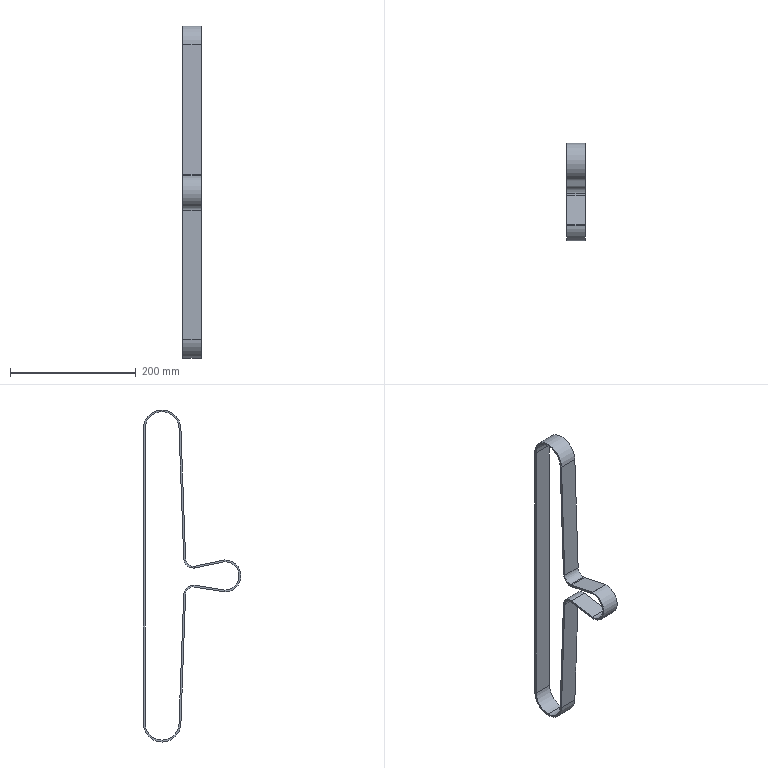Component | SolidWorks | Belt-1 | 1 solid | 28 faces | box 30 x 155.5 x 528 mm | volume 115040 mm3 | cylinder 16 | plane 12 | commonest cylinder face diameters 31.04 x3 54 x3 60 x3 25.04 x3 51 x3 45 x1
build123d program:
from build123d import *

# Parameters (mm, degrees)
BOSS_EXTRUDE1_DEPTH = 15


with BuildPart() as part:
    # Sketch1 → Boss-Extrude1 (new, symmetric)
    with BuildSketch(Plane.XY):
        with BuildLine():
            Line((-104.56, 30), (363.44, 30))
            ThreePointArc((363.44, 30), (393.44, 0.03848), (363.517, -30))
            Line((363.517, -30), (156.987, -37.488))
            ThreePointArc((156.987, -37.488), (147.591, -42.27), (145.179, -52.533))
            Line((145.179, -52.533), (154.939, -99.785))
            ThreePointArc((154.939, -99.785), (129.473, -125.5), (103.941, -99.851))
            Line((103.941, -99.851), (111.795, -52.029))
            ThreePointArc((111.795, -52.029), (109.13, -42.072), (99.898, -37.488))
            Line((99.898, -37.488), (-104.639, -30))
            ThreePointArc((-104.639, -30), (-134.56, 0.03959), (-104.56, 30))
        make_face()
        with BuildLine():
            Line((-104.56, 27), (363.44, 27))
            ThreePointArc((363.44, 27), (390.44, 0), (363.44, -27))
            Line((363.44, -27), (156.878, -34.49))
            ThreePointArc((156.878, -34.49), (145.229, -40.42), (142.242, -53.146))
            Line((142.242, -53.146), (151.94, -100))
            ThreePointArc((151.94, -100), (129.44, -122.5), (106.94, -100))
            Line((106.94, -100), (114.754, -52.52))
            ThreePointArc((114.754, -52.52), (111.454, -40.174), (100.008, -34.49))
            Line((100.008, -34.49), (-104.56, -27))
            ThreePointArc((-104.56, -27), (-131.56, 0), (-104.56, 27))
        make_face(mode=Mode.SUBTRACT)
    extrude(amount=BOSS_EXTRUDE1_DEPTH, both=True)


solid = part.part

# Placed as in the assembly
solid = solid.moved(Location((-0.0005, 4.001, -329.44), (0, -90, 0)))
STEP:
#1=COLOUR_RGB('',0.7922,0.8196,0.9333);
#2=FILL_AREA_STYLE_COLOUR('',#1);
#3=FILL_AREA_STYLE('',(#2));
#4=SURFACE_STYLE_FILL_AREA(#3);
#5=SURFACE_SIDE_STYLE('',(#4));
#6=SURFACE_STYLE_USAGE(.BOTH.,#5);
#7=PRESENTATION_STYLE_ASSIGNMENT((#6));
#8=CARTESIAN_POINT('',(-0.5906,-1.935,-7.37));
#9=VERTEX_POINT('',#8);
#10=CARTESIAN_POINT('',(-0.5906,-1.811,-7.383));
#11=VERTEX_POINT('',#10);
#12=CARTESIAN_POINT('',(-0.5906,-1.811,-6.772));
#13=DIRECTION('',(1.,0.,0.));
#14=DIRECTION('',(0.,0.,-1.));
#15=AXIS2_PLACEMENT_3D('',#12,#13,#14);
#16=CIRCLE('',#15,0.611);
#17=EDGE_CURVE('',#9,#11,#16,.T.);
#18=ORIENTED_EDGE('',*,*,#17,.T.);
#19=CARTESIAN_POINT('',(0.5905,-1.811,-7.383));
#20=VERTEX_POINT('',#19);
#21=CARTESIAN_POINT('',(-0.5906,-1.811,-7.383));
#22=DIRECTION('',(1.,0.,0.));
#23=VECTOR('',#22,39.37);
#24=LINE('',#21,#23);
#25=EDGE_CURVE('',#11,#20,#24,.T.);
#26=ORIENTED_EDGE('',*,*,#25,.T.);
#27=CARTESIAN_POINT('',(0.5905,-1.935,-7.37));
#28=VERTEX_POINT('',#27);
#29=CARTESIAN_POINT('',(0.5905,-1.811,-6.772));
#30=DIRECTION('',(1.,0.,0.));
#31=DIRECTION('',(0.,0.,-1.));
#32=AXIS2_PLACEMENT_3D('',#29,#30,#31);
#33=CIRCLE('',#32,0.611);
#34=EDGE_CURVE('',#28,#20,#33,.T.);
#35=ORIENTED_EDGE('',*,*,#34,.F.);
#36=CARTESIAN_POINT('',(-0.5906,-1.935,-7.37));
#37=DIRECTION('',(1.,0.,0.));
#38=VECTOR('',#37,39.37);
#39=LINE('',#36,#38);
#40=EDGE_CURVE('',#9,#28,#39,.T.);
#41=ORIENTED_EDGE('',*,*,#40,.F.);
#42=EDGE_LOOP('',(#18,#26,#35,#41));
#43=FACE_OUTER_BOUND('',#42,.T.);
#44=CARTESIAN_POINT('',(-0.5906,-1.811,-6.772));
#45=DIRECTION('',(1.,0.,0.));
#46=DIRECTION('',(0.,0.,-1.));
#47=AXIS2_PLACEMENT_3D('',#44,#45,#46);
#48=CYLINDRICAL_SURFACE('',#47,0.611);
#49=ADVANCED_FACE('',(#43),#48,.T.);
#50=CARTESIAN_POINT('',(-0.5906,1.221,-17.087));
#51=VERTEX_POINT('',#50);
#52=CARTESIAN_POINT('',(-0.5906,0.1575,-18.15));
#53=VERTEX_POINT('',#52);
#54=CARTESIAN_POINT('',(-0.5906,0.1575,-17.087));
#55=DIRECTION('',(-1.,0.,0.));
#56=DIRECTION('',(0.,0.,1.));
#57=AXIS2_PLACEMENT_3D('',#54,#55,#56);
#58=CIRCLE('',#57,1.063);
#59=EDGE_CURVE('',#51,#53,#58,.T.);
#60=ORIENTED_EDGE('',*,*,#59,.T.);
#61=CARTESIAN_POINT('',(0.5905,0.1575,-18.15));
#62=VERTEX_POINT('',#61);
#63=CARTESIAN_POINT('',(-0.5906,0.1575,-18.15));
#64=DIRECTION('',(1.,0.,0.));
#65=VECTOR('',#64,39.37);
#66=LINE('',#63,#65);
#67=EDGE_CURVE('',#53,#62,#66,.T.);
#68=ORIENTED_EDGE('',*,*,#67,.T.);
#69=CARTESIAN_POINT('',(0.5905,1.221,-17.087));
#70=VERTEX_POINT('',#69);
#71=CARTESIAN_POINT('',(0.5905,0.1575,-17.087));
#72=DIRECTION('',(-1.,0.,0.));
#73=DIRECTION('',(0.,0.,1.));
#74=AXIS2_PLACEMENT_3D('',#71,#72,#73);
#75=CIRCLE('',#74,1.063);
#76=EDGE_CURVE('',#70,#62,#75,.T.);
#77=ORIENTED_EDGE('',*,*,#76,.F.);
#78=CARTESIAN_POINT('',(-0.5906,1.221,-17.087));
#79=DIRECTION('',(1.,0.,0.));
#80=VECTOR('',#79,39.37);
#81=LINE('',#78,#80);
#82=EDGE_CURVE('',#51,#70,#81,.T.);
#83=ORIENTED_EDGE('',*,*,#82,.F.);
#84=EDGE_LOOP('',(#60,#68,#77,#83));
#85=FACE_OUTER_BOUND('',#84,.T.);
#86=CARTESIAN_POINT('',(-0.5906,0.1575,-17.087));
#87=DIRECTION('',(1.,0.,0.));
#88=DIRECTION('',(0.,0.,-1.));
#89=AXIS2_PLACEMENT_3D('',#86,#87,#88);
#90=CYLINDRICAL_SURFACE('',#89,1.063);
#91=ADVANCED_FACE('',(#85),#90,.F.);
#92=CARTESIAN_POINT('',(-0.5906,0.1575,-18.268));
#93=VERTEX_POINT('',#92);
#94=CARTESIAN_POINT('',(-0.5906,-1.024,-17.09));
#95=VERTEX_POINT('',#94);
#96=CARTESIAN_POINT('',(-0.5906,0.1575,-17.087));
#97=DIRECTION('',(-1.,0.,0.));
#98=DIRECTION('',(0.,0.,1.));
#99=AXIS2_PLACEMENT_3D('',#96,#97,#98);
#100=CIRCLE('',#99,1.181);
#101=EDGE_CURVE('',#93,#95,#100,.T.);
#102=ORIENTED_EDGE('',*,*,#101,.F.);
#103=CARTESIAN_POINT('',(0.5905,0.1575,-18.268));
#104=VERTEX_POINT('',#103);
#105=CARTESIAN_POINT('',(-0.5906,0.1575,-18.268));
#106=DIRECTION('',(1.,0.,0.));
#107=VECTOR('',#106,39.37);
#108=LINE('',#105,#107);
#109=EDGE_CURVE('',#93,#104,#108,.T.);
#110=ORIENTED_EDGE('',*,*,#109,.T.);
#111=CARTESIAN_POINT('',(0.5905,-1.024,-17.09));
#112=VERTEX_POINT('',#111);
#113=CARTESIAN_POINT('',(0.5905,0.1575,-17.087));
#114=DIRECTION('',(-1.,0.,0.));
#115=DIRECTION('',(0.,0.,1.));
#116=AXIS2_PLACEMENT_3D('',#113,#114,#115);
#117=CIRCLE('',#116,1.181);
#118=EDGE_CURVE('',#104,#112,#117,.T.);
#119=ORIENTED_EDGE('',*,*,#118,.T.);
#120=CARTESIAN_POINT('',(-0.5906,-1.024,-17.09));
#121=DIRECTION('',(1.,0.,0.));
#122=VECTOR('',#121,39.37);
#123=LINE('',#120,#122);
#124=EDGE_CURVE('',#95,#112,#123,.T.);
#125=ORIENTED_EDGE('',*,*,#124,.F.);
#126=EDGE_LOOP('',(#102,#110,#119,#125));
#127=FACE_OUTER_BOUND('',#126,.T.);
#128=CARTESIAN_POINT('',(-0.5906,0.1575,-17.087));
#129=DIRECTION('',(1.,0.,0.));
#130=DIRECTION('',(0.,0.,-1.));
#131=AXIS2_PLACEMENT_3D('',#128,#129,#130);
#132=CYLINDRICAL_SURFACE('',#131,1.181);
#133=ADVANCED_FACE('',(#127),#132,.T.);
#134=CARTESIAN_POINT('',(-0.5906,-1.811,-7.265));
#135=VERTEX_POINT('',#134);
#136=CARTESIAN_POINT('',(-0.5906,-1.318,-6.79));
#137=VERTEX_POINT('',#136);
#138=CARTESIAN_POINT('',(-0.5906,-1.811,-6.772));
#139=DIRECTION('',(1.,0.,0.));
#140=DIRECTION('',(0.,0.,-1.));
#141=AXIS2_PLACEMENT_3D('',#138,#139,#140);
#142=CIRCLE('',#141,0.4929);
#143=EDGE_CURVE('',#135,#137,#142,.T.);
#144=ORIENTED_EDGE('',*,*,#143,.F.);
#145=CARTESIAN_POINT('',(0.5905,-1.811,-7.265));
#146=VERTEX_POINT('',#145);
#147=CARTESIAN_POINT('',(-0.5906,-1.811,-7.265));
#148=DIRECTION('',(1.,0.,0.));
#149=VECTOR('',#148,39.37);
#150=LINE('',#147,#149);
#151=EDGE_CURVE('',#135,#146,#150,.T.);
#152=ORIENTED_EDGE('',*,*,#151,.T.);
#153=CARTESIAN_POINT('',(0.5905,-1.318,-6.79));
#154=VERTEX_POINT('',#153);
#155=CARTESIAN_POINT('',(0.5905,-1.811,-6.772));
#156=DIRECTION('',(1.,0.,0.));
#157=DIRECTION('',(0.,0.,-1.));
#158=AXIS2_PLACEMENT_3D('',#155,#156,#157);
#159=CIRCLE('',#158,0.4929);
#160=EDGE_CURVE('',#146,#154,#159,.T.);
#161=ORIENTED_EDGE('',*,*,#160,.T.);
#162=CARTESIAN_POINT('',(-0.5906,-1.318,-6.79));
#163=DIRECTION('',(1.,0.,0.));
#164=VECTOR('',#163,39.37);
#165=LINE('',#162,#164);
#166=EDGE_CURVE('',#137,#154,#165,.T.);
#167=ORIENTED_EDGE('',*,*,#166,.F.);
#168=EDGE_LOOP('',(#144,#152,#161,#167));
#169=FACE_OUTER_BOUND('',#168,.T.);
#170=CARTESIAN_POINT('',(-0.5906,-1.811,-6.772));
#171=DIRECTION('',(1.,0.,0.));
#172=DIRECTION('',(0.,0.,-1.));
#173=AXIS2_PLACEMENT_3D('',#170,#171,#172);
#174=CYLINDRICAL_SURFACE('',#173,0.4929);
#175=ADVANCED_FACE('',(#169),#174,.F.);
#176=CARTESIAN_POINT('',(-0.5906,-3.779,-6.87));
#177=VERTEX_POINT('',#176);
#178=CARTESIAN_POINT('',(-0.5906,-3.771,-6.87));
#179=VERTEX_POINT('',#178);
#180=CARTESIAN_POINT('',(-0.5906,-3.779,-7.874));
#181=DIRECTION('',(-1.,0.,0.));
#182=DIRECTION('',(0.,0.,1.));
#183=AXIS2_PLACEMENT_3D('',#180,#181,#182);
#184=CIRCLE('',#183,1.004);
#185=EDGE_CURVE('',#177,#179,#184,.T.);
#186=ORIENTED_EDGE('',*,*,#185,.F.);
#187=CARTESIAN_POINT('',(0.5905,-3.779,-6.87));
#188=VERTEX_POINT('',#187);
#189=CARTESIAN_POINT('',(-0.5906,-3.779,-6.87));
#190=DIRECTION('',(1.,0.,0.));
#191=VECTOR('',#190,39.37);
#192=LINE('',#189,#191);
#193=EDGE_CURVE('',#177,#188,#192,.T.);
#194=ORIENTED_EDGE('',*,*,#193,.T.);
#195=CARTESIAN_POINT('',(0.5905,-3.771,-6.87));
#196=VERTEX_POINT('',#195);
#197=CARTESIAN_POINT('',(0.5905,-3.779,-7.874));
#198=DIRECTION('',(-1.,0.,0.));
#199=DIRECTION('',(0.,0.,1.));
#200=AXIS2_PLACEMENT_3D('',#197,#198,#199);
#201=CIRCLE('',#200,1.004);
#202=EDGE_CURVE('',#188,#196,#201,.T.);
#203=ORIENTED_EDGE('',*,*,#202,.T.);
#204=CARTESIAN_POINT('',(-0.5906,-3.771,-6.87));
#205=DIRECTION('',(1.,0.,0.));
#206=VECTOR('',#205,39.37);
#207=LINE('',#204,#206);
#208=EDGE_CURVE('',#179,#196,#207,.T.);
#209=ORIENTED_EDGE('',*,*,#208,.F.);
#210=EDGE_LOOP('',(#186,#194,#203,#209));
#211=FACE_OUTER_BOUND('',#210,.T.);
#212=CARTESIAN_POINT('',(-0.5906,-3.779,-7.874));
#213=DIRECTION('',(1.,0.,0.));
#214=DIRECTION('',(0.,0.,-1.));
#215=AXIS2_PLACEMENT_3D('',#212,#213,#214);
#216=CYLINDRICAL_SURFACE('',#215,1.004);
#217=ADVANCED_FACE('',(#211),#216,.T.);
#218=ORIENTED_EDGE('',*,*,#193,.F.);
#219=CARTESIAN_POINT('',(-0.5906,-3.779,-8.878));
#220=VERTEX_POINT('',#219);
#221=CARTESIAN_POINT('',(-0.5906,-3.779,-7.874));
#222=DIRECTION('',(-1.,0.,0.));
#223=DIRECTION('',(0.,0.,1.));
#224=AXIS2_PLACEMENT_3D('',#221,#222,#223);
#225=CIRCLE('',#224,1.004);
#226=EDGE_CURVE('',#220,#177,#225,.T.);
#227=ORIENTED_EDGE('',*,*,#226,.F.);
#228=CARTESIAN_POINT('',(0.5905,-3.779,-8.878));
#229=VERTEX_POINT('',#228);
#230=CARTESIAN_POINT('',(-0.5906,-3.779,-8.878));
#231=DIRECTION('',(1.,0.,0.));
#232=VECTOR('',#231,39.37);
#233=LINE('',#230,#232);
#234=EDGE_CURVE('',#220,#229,#233,.T.);
#235=ORIENTED_EDGE('',*,*,#234,.T.);
#236=CARTESIAN_POINT('',(0.5905,-3.779,-7.874));
#237=DIRECTION('',(-1.,0.,0.));
#238=DIRECTION('',(0.,0.,1.));
#239=AXIS2_PLACEMENT_3D('',#236,#237,#238);
#240=CIRCLE('',#239,1.004);
#241=EDGE_CURVE('',#229,#188,#240,.T.);
#242=ORIENTED_EDGE('',*,*,#241,.T.);
#243=EDGE_LOOP('',(#218,#227,#235,#242));
#244=FACE_OUTER_BOUND('',#243,.T.);
#245=CARTESIAN_POINT('',(-0.5906,-3.779,-7.874));
#246=DIRECTION('',(1.,0.,0.));
#247=DIRECTION('',(0.,0.,-1.));
#248=AXIS2_PLACEMENT_3D('',#245,#246,#247);
#249=CYLINDRICAL_SURFACE('',#248,1.004);
#250=ADVANCED_FACE('',(#244),#249,.T.);
#251=CARTESIAN_POINT('',(-0.5906,-3.774,-8.878));
#252=VERTEX_POINT('',#251);
#253=CARTESIAN_POINT('',(-0.5906,-3.779,-7.874));
#254=DIRECTION('',(-1.,0.,0.));
#255=DIRECTION('',(0.,0.,1.));
#256=AXIS2_PLACEMENT_3D('',#253,#254,#255);
#257=CIRCLE('',#256,1.004);
#258=EDGE_CURVE('',#252,#220,#257,.T.);
#259=ORIENTED_EDGE('',*,*,#258,.T.);
#260=ORIENTED_EDGE('',*,*,#226,.T.);
#261=ORIENTED_EDGE('',*,*,#185,.T.);
#262=CARTESIAN_POINT('',(-0.5906,-1.911,-7.254));
#263=VERTEX_POINT('',#262);
#264=CARTESIAN_POINT('',(-0.5906,-3.771,-6.87));
#265=DIRECTION('',(0.,0.9793,-0.2023));
#266=VECTOR('',#265,39.37);
#267=LINE('',#264,#266);
#268=EDGE_CURVE('',#179,#263,#267,.T.);
#269=ORIENTED_EDGE('',*,*,#268,.T.);
#270=CARTESIAN_POINT('',(-0.5906,-1.811,-6.772));
#271=DIRECTION('',(1.,0.,0.));
#272=DIRECTION('',(0.,0.,-1.));
#273=AXIS2_PLACEMENT_3D('',#270,#271,#272);
#274=CIRCLE('',#273,0.4929);
#275=EDGE_CURVE('',#263,#135,#274,.T.);
#276=ORIENTED_EDGE('',*,*,#275,.T.);
#277=ORIENTED_EDGE('',*,*,#143,.T.);
#278=CARTESIAN_POINT('',(-0.5906,-1.024,1.342));
#279=VERTEX_POINT('',#278);
#280=CARTESIAN_POINT('',(-0.5906,-1.024,1.342));
#281=DIRECTION('',(0.,0.03623,0.9993));
#282=VECTOR('',#281,39.37);
#283=LINE('',#280,#282);
#284=EDGE_CURVE('',#137,#279,#283,.T.);
#285=ORIENTED_EDGE('',*,*,#284,.T.);
#286=CARTESIAN_POINT('',(-0.5906,1.339,1.339));
#287=VERTEX_POINT('',#286);
#288=CARTESIAN_POINT('',(-0.5906,0.1575,1.339));
#289=DIRECTION('',(-1.,0.,0.));
#290=DIRECTION('',(0.,0.,-1.));
#291=AXIS2_PLACEMENT_3D('',#288,#289,#290);
#292=CIRCLE('',#291,1.181);
#293=EDGE_CURVE('',#279,#287,#292,.T.);
#294=ORIENTED_EDGE('',*,*,#293,.T.);
#295=CARTESIAN_POINT('',(-0.5906,1.339,-17.087));
#296=VERTEX_POINT('',#295);
#297=CARTESIAN_POINT('',(-0.5906,1.339,-17.087));
#298=DIRECTION('',(0.,-0.,-1.));
#299=VECTOR('',#298,39.37);
#300=LINE('',#297,#299);
#301=EDGE_CURVE('',#287,#296,#300,.T.);
#302=ORIENTED_EDGE('',*,*,#301,.T.);
#303=CARTESIAN_POINT('',(-0.5906,0.1575,-17.087));
#304=DIRECTION('',(-1.,0.,0.));
#305=DIRECTION('',(0.,0.,1.));
#306=AXIS2_PLACEMENT_3D('',#303,#304,#305);
#307=CIRCLE('',#306,1.181);
#308=EDGE_CURVE('',#296,#93,#307,.T.);
#309=ORIENTED_EDGE('',*,*,#308,.T.);
#310=ORIENTED_EDGE('',*,*,#101,.T.);
#311=CARTESIAN_POINT('',(-0.5906,-1.318,-9.037));
#312=VERTEX_POINT('',#311);
#313=CARTESIAN_POINT('',(-0.5906,-1.024,-17.09));
#314=DIRECTION('',(0.,-0.03659,0.9993));
#315=VECTOR('',#314,39.37);
#316=LINE('',#313,#315);
#317=EDGE_CURVE('',#95,#312,#316,.T.);
#318=ORIENTED_EDGE('',*,*,#317,.T.);
#319=CARTESIAN_POINT('',(-0.5906,-1.891,-8.569));
#320=VERTEX_POINT('',#319);
#321=CARTESIAN_POINT('',(-0.5906,-1.811,-9.055));
#322=DIRECTION('',(1.,0.,0.));
#323=DIRECTION('',(0.,0.,-1.));
#324=AXIS2_PLACEMENT_3D('',#321,#322,#323);
#325=CIRCLE('',#324,0.4929);
#326=EDGE_CURVE('',#312,#320,#325,.T.);
#327=ORIENTED_EDGE('',*,*,#326,.T.);
#328=CARTESIAN_POINT('',(-0.5906,-3.774,-8.878));
#329=DIRECTION('',(0.,-0.9868,-0.1621));
#330=VECTOR('',#329,39.37);
#331=LINE('',#328,#330);
#332=EDGE_CURVE('',#320,#252,#331,.T.);
#333=ORIENTED_EDGE('',*,*,#332,.T.);
#334=EDGE_LOOP('',(#259,#260,#261,#269,#276,#277,#285,#294,#302,#309,#310,#318,#327,#333));
#335=FACE_OUTER_BOUND('',#334,.T.);
#336=CARTESIAN_POINT('',(-0.5906,-0.9055,-17.087));
#337=VERTEX_POINT('',#336);
#338=CARTESIAN_POINT('',(-0.5906,-1.2,-9.033));
#339=VERTEX_POINT('',#338);
#340=CARTESIAN_POINT('',(-0.5906,-0.9055,-17.087));
#341=DIRECTION('',(0.,-0.03659,0.9993));
#342=VECTOR('',#341,39.37);
#343=LINE('',#340,#342);
#344=EDGE_CURVE('',#337,#339,#343,.T.);
#345=ORIENTED_EDGE('',*,*,#344,.F.);
#346=CARTESIAN_POINT('',(-0.5906,0.1575,-17.087));
#347=DIRECTION('',(-1.,0.,0.));
#348=DIRECTION('',(0.,0.,1.));
#349=AXIS2_PLACEMENT_3D('',#346,#347,#348);
#350=CIRCLE('',#349,1.063);
#351=EDGE_CURVE('',#53,#337,#350,.T.);
#352=ORIENTED_EDGE('',*,*,#351,.F.);
#353=ORIENTED_EDGE('',*,*,#59,.F.);
#354=CARTESIAN_POINT('',(-0.5906,1.221,1.339));
#355=VERTEX_POINT('',#354);
#356=CARTESIAN_POINT('',(-0.5906,1.221,-17.087));
#357=DIRECTION('',(0.,0.,-1.));
#358=VECTOR('',#357,39.37);
#359=LINE('',#356,#358);
#360=EDGE_CURVE('',#355,#51,#359,.T.);
#361=ORIENTED_EDGE('',*,*,#360,.F.);
#362=CARTESIAN_POINT('',(-0.5906,-0.9055,1.339));
#363=VERTEX_POINT('',#362);
#364=CARTESIAN_POINT('',(-0.5906,0.1575,1.339));
#365=DIRECTION('',(-1.,0.,0.));
#366=DIRECTION('',(0.,0.,-1.));
#367=AXIS2_PLACEMENT_3D('',#364,#365,#366);
#368=CIRCLE('',#367,1.063);
#369=EDGE_CURVE('',#363,#355,#368,.T.);
#370=ORIENTED_EDGE('',*,*,#369,.F.);
#371=CARTESIAN_POINT('',(-0.5906,-1.2,-6.794));
#372=VERTEX_POINT('',#371);
#373=CARTESIAN_POINT('',(-0.5906,-0.9055,1.339));
#374=DIRECTION('',(0.,0.03624,0.9993));
#375=VECTOR('',#374,39.37);
#376=LINE('',#373,#375);
#377=EDGE_CURVE('',#372,#363,#376,.T.);
#378=ORIENTED_EDGE('',*,*,#377,.F.);
#379=CARTESIAN_POINT('',(-0.5906,-1.811,-6.772));
#380=DIRECTION('',(1.,0.,0.));
#381=DIRECTION('',(0.,0.,-1.));
#382=AXIS2_PLACEMENT_3D('',#379,#380,#381);
#383=CIRCLE('',#382,0.611);
#384=EDGE_CURVE('',#11,#372,#383,.T.);
#385=ORIENTED_EDGE('',*,*,#384,.F.);
#386=ORIENTED_EDGE('',*,*,#17,.F.);
#387=CARTESIAN_POINT('',(-0.5906,-3.779,-6.988));
#388=VERTEX_POINT('',#387);
#389=CARTESIAN_POINT('',(-0.5906,-3.779,-6.988));
#390=DIRECTION('',(0.,0.9792,-0.2027));
#391=VECTOR('',#390,39.37);
#392=LINE('',#389,#391);
#393=EDGE_CURVE('',#388,#9,#392,.T.);
#394=ORIENTED_EDGE('',*,*,#393,.F.);
#395=CARTESIAN_POINT('',(-0.5906,-3.779,-8.76));
#396=VERTEX_POINT('',#395);
#397=CARTESIAN_POINT('',(-0.5906,-3.779,-7.874));
#398=DIRECTION('',(-1.,0.,0.));
#399=DIRECTION('',(0.,0.,1.));
#400=AXIS2_PLACEMENT_3D('',#397,#398,#399);
#401=CIRCLE('',#400,0.8858);
#402=EDGE_CURVE('',#396,#388,#401,.T.);
#403=ORIENTED_EDGE('',*,*,#402,.F.);
#404=CARTESIAN_POINT('',(-0.5906,-1.91,-8.452));
#405=VERTEX_POINT('',#404);
#406=CARTESIAN_POINT('',(-0.5906,-3.779,-8.76));
#407=DIRECTION('',(0.,-0.9867,-0.1624));
#408=VECTOR('',#407,39.37);
#409=LINE('',#406,#408);
#410=EDGE_CURVE('',#405,#396,#409,.T.);
#411=ORIENTED_EDGE('',*,*,#410,.F.);
#412=CARTESIAN_POINT('',(-0.5906,-1.811,-9.055));
#413=DIRECTION('',(1.,0.,0.));
#414=DIRECTION('',(0.,0.,-1.));
#415=AXIS2_PLACEMENT_3D('',#412,#413,#414);
#416=CIRCLE('',#415,0.611);
#417=EDGE_CURVE('',#339,#405,#416,.T.);
#418=ORIENTED_EDGE('',*,*,#417,.F.);
#419=EDGE_LOOP('',(#345,#352,#353,#361,#370,#378,#385,#386,#394,#403,#411,#418));
#420=FACE_BOUND('',#419,.T.);
#421=CARTESIAN_POINT('',(-0.5906,-3.779,-7.874));
#422=DIRECTION('',(-1.,0.,0.));
#423=DIRECTION('',(0.,0.,1.));
#424=AXIS2_PLACEMENT_3D('',#421,#422,#423);
#425=PLANE('',#424);
#426=ADVANCED_FACE('',(#335,#420),#425,.T.);
#427=CARTESIAN_POINT('',(0.5905,-3.774,-8.878));
#428=VERTEX_POINT('',#427);
#429=CARTESIAN_POINT('',(0.5905,-3.779,-7.874));
#430=DIRECTION('',(-1.,0.,0.));
#431=DIRECTION('',(0.,0.,1.));
#432=AXIS2_PLACEMENT_3D('',#429,#430,#431);
#433=CIRCLE('',#432,1.004);
#434=EDGE_CURVE('',#428,#229,#433,.T.);
#435=ORIENTED_EDGE('',*,*,#434,.F.);
#436=CARTESIAN_POINT('',(0.5905,-1.891,-8.569));
#437=VERTEX_POINT('',#436);
#438=CARTESIAN_POINT('',(0.5905,-3.774,-8.878));
#439=DIRECTION('',(0.,-0.9868,-0.1621));
#440=VECTOR('',#439,39.37);
#441=LINE('',#438,#440);
#442=EDGE_CURVE('',#437,#428,#441,.T.);
#443=ORIENTED_EDGE('',*,*,#442,.F.);
#444=CARTESIAN_POINT('',(0.5905,-1.318,-9.037));
#445=VERTEX_POINT('',#444);
#446=CARTESIAN_POINT('',(0.5905,-1.811,-9.055));
#447=DIRECTION('',(1.,0.,0.));
#448=DIRECTION('',(0.,0.,-1.));
#449=AXIS2_PLACEMENT_3D('',#446,#447,#448);
#450=CIRCLE('',#449,0.4929);
#451=EDGE_CURVE('',#445,#437,#450,.T.);
#452=ORIENTED_EDGE('',*,*,#451,.F.);
#453=CARTESIAN_POINT('',(0.5905,-1.024,-17.09));
#454=DIRECTION('',(0.,-0.03659,0.9993));
#455=VECTOR('',#454,39.37);
#456=LINE('',#453,#455);
#457=EDGE_CURVE('',#112,#445,#456,.T.);
#458=ORIENTED_EDGE('',*,*,#457,.F.);
#459=ORIENTED_EDGE('',*,*,#118,.F.);
#460=CARTESIAN_POINT('',(0.5905,1.339,-17.087));
#461=VERTEX_POINT('',#460);
#462=CARTESIAN_POINT('',(0.5905,0.1575,-17.087));
#463=DIRECTION('',(-1.,0.,0.));
#464=DIRECTION('',(0.,0.,1.));
#465=AXIS2_PLACEMENT_3D('',#462,#463,#464);
#466=CIRCLE('',#465,1.181);
#467=EDGE_CURVE('',#461,#104,#466,.T.);
#468=ORIENTED_EDGE('',*,*,#467,.F.);
#469=CARTESIAN_POINT('',(0.5905,1.339,1.339));
#470=VERTEX_POINT('',#469);
#471=CARTESIAN_POINT('',(0.5905,1.339,-17.087));
#472=DIRECTION('',(0.,-0.,-1.));
#473=VECTOR('',#472,39.37);
#474=LINE('',#471,#473);
#475=EDGE_CURVE('',#470,#461,#474,.T.);
#476=ORIENTED_EDGE('',*,*,#475,.F.);
#477=CARTESIAN_POINT('',(0.5905,-1.024,1.342));
#478=VERTEX_POINT('',#477);
#479=CARTESIAN_POINT('',(0.5905,0.1575,1.339));
#480=DIRECTION('',(-1.,0.,0.));
#481=DIRECTION('',(0.,0.,-1.));
#482=AXIS2_PLACEMENT_3D('',#479,#480,#481);
#483=CIRCLE('',#482,1.181);
#484=EDGE_CURVE('',#478,#470,#483,.T.);
#485=ORIENTED_EDGE('',*,*,#484,.F.);
#486=CARTESIAN_POINT('',(0.5905,-1.024,1.342));
#487=DIRECTION('',(0.,0.03623,0.9993));
#488=VECTOR('',#487,39.37);
#489=LINE('',#486,#488);
#490=EDGE_CURVE('',#154,#478,#489,.T.);
#491=ORIENTED_EDGE('',*,*,#490,.F.);
#492=ORIENTED_EDGE('',*,*,#160,.F.);
#493=CARTESIAN_POINT('',(0.5905,-1.911,-7.254));
#494=VERTEX_POINT('',#493);
#495=CARTESIAN_POINT('',(0.5905,-1.811,-6.772));
#496=DIRECTION('',(1.,0.,0.));
#497=DIRECTION('',(0.,0.,-1.));
#498=AXIS2_PLACEMENT_3D('',#495,#496,#497);
#499=CIRCLE('',#498,0.4929);
#500=EDGE_CURVE('',#494,#146,#499,.T.);
#501=ORIENTED_EDGE('',*,*,#500,.F.);
#502=CARTESIAN_POINT('',(0.5905,-3.771,-6.87));
#503=DIRECTION('',(0.,0.9793,-0.2023));
#504=VECTOR('',#503,39.37);
#505=LINE('',#502,#504);
#506=EDGE_CURVE('',#196,#494,#505,.T.);
#507=ORIENTED_EDGE('',*,*,#506,.F.);
#508=ORIENTED_EDGE('',*,*,#202,.F.);
#509=ORIENTED_EDGE('',*,*,#241,.F.);
#510=EDGE_LOOP('',(#435,#443,#452,#458,#459,#468,#476,#485,#491,#492,#501,#507,#508,#509));
#511=FACE_OUTER_BOUND('',#510,.T.);
#512=ORIENTED_EDGE('',*,*,#76,.T.);
#513=CARTESIAN_POINT('',(0.5905,-0.9055,-17.087));
#514=VERTEX_POINT('',#513);
#515=CARTESIAN_POINT('',(0.5905,0.1575,-17.087));
#516=DIRECTION('',(-1.,0.,0.));
#517=DIRECTION('',(0.,0.,1.));
#518=AXIS2_PLACEMENT_3D('',#515,#516,#517);
#519=CIRCLE('',#518,1.063);
#520=EDGE_CURVE('',#62,#514,#519,.T.);
#521=ORIENTED_EDGE('',*,*,#520,.T.);
#522=CARTESIAN_POINT('',(0.5905,-1.2,-9.033));
#523=VERTEX_POINT('',#522);
#524=CARTESIAN_POINT('',(0.5905,-0.9055,-17.087));
#525=DIRECTION('',(0.,-0.03659,0.9993));
#526=VECTOR('',#525,39.37);
#527=LINE('',#524,#526);
#528=EDGE_CURVE('',#514,#523,#527,.T.);
#529=ORIENTED_EDGE('',*,*,#528,.T.);
#530=CARTESIAN_POINT('',(0.5905,-1.91,-8.452));
#531=VERTEX_POINT('',#530);
#532=CARTESIAN_POINT('',(0.5905,-1.811,-9.055));
#533=DIRECTION('',(1.,0.,0.));
#534=DIRECTION('',(0.,0.,-1.));
#535=AXIS2_PLACEMENT_3D('',#532,#533,#534);
#536=CIRCLE('',#535,0.611);
#537=EDGE_CURVE('',#523,#531,#536,.T.);
#538=ORIENTED_EDGE('',*,*,#537,.T.);
#539=CARTESIAN_POINT('',(0.5905,-3.779,-8.76));
#540=VERTEX_POINT('',#539);
#541=CARTESIAN_POINT('',(0.5905,-3.779,-8.76));
#542=DIRECTION('',(0.,-0.9867,-0.1624));
#543=VECTOR('',#542,39.37);
#544=LINE('',#541,#543);
#545=EDGE_CURVE('',#531,#540,#544,.T.);
#546=ORIENTED_EDGE('',*,*,#545,.T.);
#547=CARTESIAN_POINT('',(0.5905,-3.779,-6.988));
#548=VERTEX_POINT('',#547);
#549=CARTESIAN_POINT('',(0.5905,-3.779,-7.874));
#550=DIRECTION('',(-1.,0.,0.));
#551=DIRECTION('',(0.,0.,1.));
#552=AXIS2_PLACEMENT_3D('',#549,#550,#551);
#553=CIRCLE('',#552,0.8858);
#554=EDGE_CURVE('',#540,#548,#553,.T.);
#555=ORIENTED_EDGE('',*,*,#554,.T.);
#556=CARTESIAN_POINT('',(0.5905,-3.779,-6.988));
#557=DIRECTION('',(0.,0.9792,-0.2027));
#558=VECTOR('',#557,39.37);
#559=LINE('',#556,#558);
#560=EDGE_CURVE('',#548,#28,#559,.T.);
#561=ORIENTED_EDGE('',*,*,#560,.T.);
#562=ORIENTED_EDGE('',*,*,#34,.T.);
#563=CARTESIAN_POINT('',(0.5905,-1.2,-6.794));
#564=VERTEX_POINT('',#563);
#565=CARTESIAN_POINT('',(0.5905,-1.811,-6.772));
#566=DIRECTION('',(1.,0.,0.));
#567=DIRECTION('',(0.,0.,-1.));
#568=AXIS2_PLACEMENT_3D('',#565,#566,#567);
#569=CIRCLE('',#568,0.611);
#570=EDGE_CURVE('',#20,#564,#569,.T.);
#571=ORIENTED_EDGE('',*,*,#570,.T.);
#572=CARTESIAN_POINT('',(0.5905,-0.9055,1.339));
#573=VERTEX_POINT('',#572);
#574=CARTESIAN_POINT('',(0.5905,-0.9055,1.339));
#575=DIRECTION('',(0.,0.03624,0.9993));
#576=VECTOR('',#575,39.37);
#577=LINE('',#574,#576);
#578=EDGE_CURVE('',#564,#573,#577,.T.);
#579=ORIENTED_EDGE('',*,*,#578,.T.);
#580=CARTESIAN_POINT('',(0.5905,1.221,1.339));
#581=VERTEX_POINT('',#580);
#582=CARTESIAN_POINT('',(0.5905,0.1575,1.339));
#583=DIRECTION('',(-1.,0.,0.));
#584=DIRECTION('',(0.,0.,-1.));
#585=AXIS2_PLACEMENT_3D('',#582,#583,#584);
#586=CIRCLE('',#585,1.063);
#587=EDGE_CURVE('',#573,#581,#586,.T.);
#588=ORIENTED_EDGE('',*,*,#587,.T.);
#589=CARTESIAN_POINT('',(0.5905,1.221,-17.087));
#590=DIRECTION('',(0.,0.,-1.));
#591=VECTOR('',#590,39.37);
#592=LINE('',#589,#591);
#593=EDGE_CURVE('',#581,#70,#592,.T.);
#594=ORIENTED_EDGE('',*,*,#593,.T.);
#595=EDGE_LOOP('',(#512,#521,#529,#538,#546,#555,#561,#562,#571,#579,#588,#594));
#596=FACE_BOUND('',#595,.T.);
#597=CARTESIAN_POINT('',(0.5905,-3.779,-7.874));
#598=DIRECTION('',(-1.,0.,0.));
#599=DIRECTION('',(0.,0.,1.));
#600=AXIS2_PLACEMENT_3D('',#597,#598,#599);
#601=PLANE('',#600);
#602=ADVANCED_FACE('',(#511,#596),#601,.F.);
#603=ORIENTED_EDGE('',*,*,#234,.F.);
#604=ORIENTED_EDGE('',*,*,#258,.F.);
#605=CARTESIAN_POINT('',(-0.5906,-3.774,-8.878));
#606=DIRECTION('',(1.,0.,0.));
#607=VECTOR('',#606,39.37);
#608=LINE('',#605,#607);
#609=EDGE_CURVE('',#252,#428,#608,.T.);
#610=ORIENTED_EDGE('',*,*,#609,.T.);
#611=ORIENTED_EDGE('',*,*,#434,.T.);
#612=EDGE_LOOP('',(#603,#604,#610,#611));
#613=FACE_OUTER_BOUND('',#612,.T.);
#614=CARTESIAN_POINT('',(-0.5906,-3.779,-7.874));
#615=DIRECTION('',(1.,0.,0.));
#616=DIRECTION('',(0.,0.,-1.));
#617=AXIS2_PLACEMENT_3D('',#614,#615,#616);
#618=CYLINDRICAL_SURFACE('',#617,1.004);
#619=ADVANCED_FACE('',(#613),#618,.T.);
#620=ORIENTED_EDGE('',*,*,#506,.T.);
#621=CARTESIAN_POINT('',(-0.5906,-1.911,-7.254));
#622=DIRECTION('',(1.,0.,0.));
#623=VECTOR('',#622,39.37);
#624=LINE('',#621,#623);
#625=EDGE_CURVE('',#263,#494,#624,.T.);
#626=ORIENTED_EDGE('',*,*,#625,.F.);
#627=ORIENTED_EDGE('',*,*,#268,.F.);
#628=ORIENTED_EDGE('',*,*,#208,.T.);
#629=EDGE_LOOP('',(#620,#626,#627,#628));
#630=FACE_OUTER_BOUND('',#629,.T.);
#631=CARTESIAN_POINT('',(-0.5906,-3.771,-6.87));
#632=DIRECTION('',(0.,-0.2023,-0.9793));
#633=DIRECTION('',(0.,-0.9793,0.2023));
#634=AXIS2_PLACEMENT_3D('',#631,#632,#633);
#635=PLANE('',#634);
#636=ADVANCED_FACE('',(#630),#635,.F.);
#637=ORIENTED_EDGE('',*,*,#151,.F.);
#638=ORIENTED_EDGE('',*,*,#275,.F.);
#639=ORIENTED_EDGE('',*,*,#625,.T.);
#640=ORIENTED_EDGE('',*,*,#500,.T.);
#641=EDGE_LOOP('',(#637,#638,#639,#640));
#642=FACE_OUTER_BOUND('',#641,.T.);
#643=CARTESIAN_POINT('',(-0.5906,-1.811,-6.772));
#644=DIRECTION('',(1.,0.,0.));
#645=DIRECTION('',(0.,0.,-1.));
#646=AXIS2_PLACEMENT_3D('',#643,#644,#645);
#647=CYLINDRICAL_SURFACE('',#646,0.4929);
#648=ADVANCED_FACE('',(#642),#647,.F.);
#649=ORIENTED_EDGE('',*,*,#490,.T.);
#650=CARTESIAN_POINT('',(-0.5906,-1.024,1.342));
#651=DIRECTION('',(1.,0.,0.));
#652=VECTOR('',#651,39.37);
#653=LINE('',#650,#652);
#654=EDGE_CURVE('',#279,#478,#653,.T.);
#655=ORIENTED_EDGE('',*,*,#654,.F.);
#656=ORIENTED_EDGE('',*,*,#284,.F.);
#657=ORIENTED_EDGE('',*,*,#166,.T.);
#658=EDGE_LOOP('',(#649,#655,#656,#657));
#659=FACE_OUTER_BOUND('',#658,.T.);
#660=CARTESIAN_POINT('',(-0.5906,-1.024,1.342));
#661=DIRECTION('',(0.,0.9993,-0.03623));
#662=DIRECTION('',(0.,-0.03623,-0.9993));
#663=AXIS2_PLACEMENT_3D('',#660,#661,#662);
#664=PLANE('',#663);
#665=ADVANCED_FACE('',(#659),#664,.F.);
#666=ORIENTED_EDGE('',*,*,#484,.T.);
#667=CARTESIAN_POINT('',(-0.5906,1.339,1.339));
#668=DIRECTION('',(1.,0.,0.));
#669=VECTOR('',#668,39.37);
#670=LINE('',#667,#669);
#671=EDGE_CURVE('',#287,#470,#670,.T.);
#672=ORIENTED_EDGE('',*,*,#671,.F.);
#673=ORIENTED_EDGE('',*,*,#293,.F.);
#674=ORIENTED_EDGE('',*,*,#654,.T.);
#675=EDGE_LOOP('',(#666,#672,#673,#674));
#676=FACE_OUTER_BOUND('',#675,.T.);
#677=CARTESIAN_POINT('',(-0.5906,0.1575,1.339));
#678=DIRECTION('',(1.,0.,0.));
#679=DIRECTION('',(0.,0.,-1.));
#680=AXIS2_PLACEMENT_3D('',#677,#678,#679);
#681=CYLINDRICAL_SURFACE('',#680,1.181);
#682=ADVANCED_FACE('',(#676),#681,.T.);
#683=ORIENTED_EDGE('',*,*,#475,.T.);
#684=CARTESIAN_POINT('',(-0.5906,1.339,-17.087));
#685=DIRECTION('',(1.,0.,0.));
#686=VECTOR('',#685,39.37);
#687=LINE('',#684,#686);
#688=EDGE_CURVE('',#296,#461,#687,.T.);
#689=ORIENTED_EDGE('',*,*,#688,.F.);
#690=ORIENTED_EDGE('',*,*,#301,.F.);
#691=ORIENTED_EDGE('',*,*,#671,.T.);
#692=EDGE_LOOP('',(#683,#689,#690,#691));
#693=FACE_OUTER_BOUND('',#692,.T.);
#694=CARTESIAN_POINT('',(-0.5906,1.339,-17.087));
#695=DIRECTION('',(0.,-1.,0.));
#696=DIRECTION('',(1.,0.,0.));
#697=AXIS2_PLACEMENT_3D('',#694,#695,#696);
#698=PLANE('',#697);
#699=ADVANCED_FACE('',(#693),#698,.F.);
#700=ORIENTED_EDGE('',*,*,#109,.F.);
#701=ORIENTED_EDGE('',*,*,#308,.F.);
#702=ORIENTED_EDGE('',*,*,#688,.T.);
#703=ORIENTED_EDGE('',*,*,#467,.T.);
#704=EDGE_LOOP('',(#700,#701,#702,#703));
#705=FACE_OUTER_BOUND('',#704,.T.);
#706=CARTESIAN_POINT('',(-0.5906,0.1575,-17.087));
#707=DIRECTION('',(1.,0.,0.));
#708=DIRECTION('',(0.,0.,-1.));
#709=AXIS2_PLACEMENT_3D('',#706,#707,#708);
#710=CYLINDRICAL_SURFACE('',#709,1.181);
#711=ADVANCED_FACE('',(#705),#710,.T.);
#712=ORIENTED_EDGE('',*,*,#457,.T.);
#713=CARTESIAN_POINT('',(-0.5906,-1.318,-9.037));
#714=DIRECTION('',(1.,0.,0.));
#715=VECTOR('',#714,39.37);
#716=LINE('',#713,#715);
#717=EDGE_CURVE('',#312,#445,#716,.T.);
#718=ORIENTED_EDGE('',*,*,#717,.F.);
#719=ORIENTED_EDGE('',*,*,#317,.F.);
#720=ORIENTED_EDGE('',*,*,#124,.T.);
#721=EDGE_LOOP('',(#712,#718,#719,#720));
#722=FACE_OUTER_BOUND('',#721,.T.);
#723=CARTESIAN_POINT('',(-0.5906,-1.024,-17.09));
#724=DIRECTION('',(0.,0.9993,0.03659));
#725=DIRECTION('',(0.,0.03659,-0.9993));
#726=AXIS2_PLACEMENT_3D('',#723,#724,#725);
#727=PLANE('',#726);
#728=ADVANCED_FACE('',(#722),#727,.F.);
#729=ORIENTED_EDGE('',*,*,#451,.T.);
#730=CARTESIAN_POINT('',(-0.5906,-1.891,-8.569));
#731=DIRECTION('',(1.,0.,0.));
#732=VECTOR('',#731,39.37);
#733=LINE('',#730,#732);
#734=EDGE_CURVE('',#320,#437,#733,.T.);
#735=ORIENTED_EDGE('',*,*,#734,.F.);
#736=ORIENTED_EDGE('',*,*,#326,.F.);
#737=ORIENTED_EDGE('',*,*,#717,.T.);
#738=EDGE_LOOP('',(#729,#735,#736,#737));
#739=FACE_OUTER_BOUND('',#738,.T.);
#740=CARTESIAN_POINT('',(-0.5906,-1.811,-9.055));
#741=DIRECTION('',(1.,0.,0.));
#742=DIRECTION('',(0.,0.,-1.));
#743=AXIS2_PLACEMENT_3D('',#740,#741,#742);
#744=CYLINDRICAL_SURFACE('',#743,0.4929);
#745=ADVANCED_FACE('',(#739),#744,.F.);
#746=ORIENTED_EDGE('',*,*,#442,.T.);
#747=ORIENTED_EDGE('',*,*,#609,.F.);
#748=ORIENTED_EDGE('',*,*,#332,.F.);
#749=ORIENTED_EDGE('',*,*,#734,.T.);
#750=EDGE_LOOP('',(#746,#747,#748,#749));
#751=FACE_OUTER_BOUND('',#750,.T.);
#752=CARTESIAN_POINT('',(-0.5906,-3.774,-8.878));
#753=DIRECTION('',(0.,-0.1621,0.9868));
#754=DIRECTION('',(0.,0.9868,0.1621));
#755=AXIS2_PLACEMENT_3D('',#752,#753,#754);
#756=PLANE('',#755);
#757=ADVANCED_FACE('',(#751),#756,.F.);
#758=ORIENTED_EDGE('',*,*,#67,.F.);
#759=ORIENTED_EDGE('',*,*,#351,.T.);
#760=CARTESIAN_POINT('',(-0.5906,-0.9055,-17.087));
#761=DIRECTION('',(1.,0.,0.));
#762=VECTOR('',#761,39.37);
#763=LINE('',#760,#762);
#764=EDGE_CURVE('',#337,#514,#763,.T.);
#765=ORIENTED_EDGE('',*,*,#764,.T.);
#766=ORIENTED_EDGE('',*,*,#520,.F.);
#767=EDGE_LOOP('',(#758,#759,#765,#766));
#768=FACE_OUTER_BOUND('',#767,.T.);
#769=CARTESIAN_POINT('',(-0.5906,0.1575,-17.087));
#770=DIRECTION('',(1.,0.,0.));
#771=DIRECTION('',(0.,0.,-1.));
#772=AXIS2_PLACEMENT_3D('',#769,#770,#771);
#773=CYLINDRICAL_SURFACE('',#772,1.063);
#774=ADVANCED_FACE('',(#768),#773,.F.);
#775=ORIENTED_EDGE('',*,*,#528,.F.);
#776=ORIENTED_EDGE('',*,*,#764,.F.);
#777=ORIENTED_EDGE('',*,*,#344,.T.);
#778=CARTESIAN_POINT('',(-0.5906,-1.2,-9.033));
#779=DIRECTION('',(1.,0.,0.));
#780=VECTOR('',#779,39.37);
#781=LINE('',#778,#780);
#782=EDGE_CURVE('',#339,#523,#781,.T.);
#783=ORIENTED_EDGE('',*,*,#782,.T.);
#784=EDGE_LOOP('',(#775,#776,#777,#783));
#785=FACE_OUTER_BOUND('',#784,.T.);
#786=CARTESIAN_POINT('',(-0.5906,-0.9055,-17.087));
#787=DIRECTION('',(0.,0.9993,0.03659));
#788=DIRECTION('',(0.,0.03659,-0.9993));
#789=AXIS2_PLACEMENT_3D('',#786,#787,#788);
#790=PLANE('',#789);
#791=ADVANCED_FACE('',(#785),#790,.T.);
#792=ORIENTED_EDGE('',*,*,#537,.F.);
#793=ORIENTED_EDGE('',*,*,#782,.F.);
#794=ORIENTED_EDGE('',*,*,#417,.T.);
#795=CARTESIAN_POINT('',(-0.5906,-1.91,-8.452));
#796=DIRECTION('',(1.,0.,0.));
#797=VECTOR('',#796,39.37);
#798=LINE('',#795,#797);
#799=EDGE_CURVE('',#405,#531,#798,.T.);
#800=ORIENTED_EDGE('',*,*,#799,.T.);
#801=EDGE_LOOP('',(#792,#793,#794,#800));
#802=FACE_OUTER_BOUND('',#801,.T.);
#803=CARTESIAN_POINT('',(-0.5906,-1.811,-9.055));
#804=DIRECTION('',(1.,0.,0.));
#805=DIRECTION('',(0.,0.,-1.));
#806=AXIS2_PLACEMENT_3D('',#803,#804,#805);
#807=CYLINDRICAL_SURFACE('',#806,0.611);
#808=ADVANCED_FACE('',(#802),#807,.T.);
#809=ORIENTED_EDGE('',*,*,#545,.F.);
#810=ORIENTED_EDGE('',*,*,#799,.F.);
#811=ORIENTED_EDGE('',*,*,#410,.T.);
#812=CARTESIAN_POINT('',(-0.5906,-3.779,-8.76));
#813=DIRECTION('',(1.,0.,0.));
#814=VECTOR('',#813,39.37);
#815=LINE('',#812,#814);
#816=EDGE_CURVE('',#396,#540,#815,.T.);
#817=ORIENTED_EDGE('',*,*,#816,.T.);
#818=EDGE_LOOP('',(#809,#810,#811,#817));
#819=FACE_OUTER_BOUND('',#818,.T.);
#820=CARTESIAN_POINT('',(-0.5906,-3.779,-8.76));
#821=DIRECTION('',(0.,-0.1624,0.9867));
#822=DIRECTION('',(0.,0.9867,0.1624));
#823=AXIS2_PLACEMENT_3D('',#820,#821,#822);
#824=PLANE('',#823);
#825=ADVANCED_FACE('',(#819),#824,.T.);
#826=ORIENTED_EDGE('',*,*,#554,.F.);
#827=ORIENTED_EDGE('',*,*,#816,.F.);
#828=ORIENTED_EDGE('',*,*,#402,.T.);
#829=CARTESIAN_POINT('',(-0.5906,-3.779,-6.988));
#830=DIRECTION('',(1.,0.,0.));
#831=VECTOR('',#830,39.37);
#832=LINE('',#829,#831);
#833=EDGE_CURVE('',#388,#548,#832,.T.);
#834=ORIENTED_EDGE('',*,*,#833,.T.);
#835=EDGE_LOOP('',(#826,#827,#828,#834));
#836=FACE_OUTER_BOUND('',#835,.T.);
#837=CARTESIAN_POINT('',(-0.5906,-3.779,-7.874));
#838=DIRECTION('',(1.,0.,0.));
#839=DIRECTION('',(0.,0.,-1.));
#840=AXIS2_PLACEMENT_3D('',#837,#838,#839);
#841=CYLINDRICAL_SURFACE('',#840,0.8858);
#842=ADVANCED_FACE('',(#836),#841,.F.);
#843=ORIENTED_EDGE('',*,*,#560,.F.);
#844=ORIENTED_EDGE('',*,*,#833,.F.);
#845=ORIENTED_EDGE('',*,*,#393,.T.);
#846=ORIENTED_EDGE('',*,*,#40,.T.);
#847=EDGE_LOOP('',(#843,#844,#845,#846));
#848=FACE_OUTER_BOUND('',#847,.T.);
#849=CARTESIAN_POINT('',(-0.5906,-3.779,-6.988));
#850=DIRECTION('',(0.,-0.2027,-0.9792));
#851=DIRECTION('',(0.,-0.9792,0.2027));
#852=AXIS2_PLACEMENT_3D('',#849,#850,#851);
#853=PLANE('',#852);
#854=ADVANCED_FACE('',(#848),#853,.T.);
#855=ORIENTED_EDGE('',*,*,#25,.F.);
#856=ORIENTED_EDGE('',*,*,#384,.T.);
#857=CARTESIAN_POINT('',(-0.5906,-1.2,-6.794));
#858=DIRECTION('',(1.,0.,0.));
#859=VECTOR('',#858,39.37);
#860=LINE('',#857,#859);
#861=EDGE_CURVE('',#372,#564,#860,.T.);
#862=ORIENTED_EDGE('',*,*,#861,.T.);
#863=ORIENTED_EDGE('',*,*,#570,.F.);
#864=EDGE_LOOP('',(#855,#856,#862,#863));
#865=FACE_OUTER_BOUND('',#864,.T.);
#866=CARTESIAN_POINT('',(-0.5906,-1.811,-6.772));
#867=DIRECTION('',(1.,0.,0.));
#868=DIRECTION('',(0.,0.,-1.));
#869=AXIS2_PLACEMENT_3D('',#866,#867,#868);
#870=CYLINDRICAL_SURFACE('',#869,0.611);
#871=ADVANCED_FACE('',(#865),#870,.T.);
#872=ORIENTED_EDGE('',*,*,#578,.F.);
#873=ORIENTED_EDGE('',*,*,#861,.F.);
#874=ORIENTED_EDGE('',*,*,#377,.T.);
#875=CARTESIAN_POINT('',(-0.5906,-0.9055,1.339));
#876=DIRECTION('',(1.,0.,0.));
#877=VECTOR('',#876,39.37);
#878=LINE('',#875,#877);
#879=EDGE_CURVE('',#363,#573,#878,.T.);
#880=ORIENTED_EDGE('',*,*,#879,.T.);
#881=EDGE_LOOP('',(#872,#873,#874,#880));
#882=FACE_OUTER_BOUND('',#881,.T.);
#883=CARTESIAN_POINT('',(-0.5906,-0.9055,1.339));
#884=DIRECTION('',(0.,0.9993,-0.03624));
#885=DIRECTION('',(0.,-0.03624,-0.9993));
#886=AXIS2_PLACEMENT_3D('',#883,#884,#885);
#887=PLANE('',#886);
#888=ADVANCED_FACE('',(#882),#887,.T.);
#889=ORIENTED_EDGE('',*,*,#587,.F.);
#890=ORIENTED_EDGE('',*,*,#879,.F.);
#891=ORIENTED_EDGE('',*,*,#369,.T.);
#892=CARTESIAN_POINT('',(-0.5906,1.221,1.339));
#893=DIRECTION('',(1.,0.,0.));
#894=VECTOR('',#893,39.37);
#895=LINE('',#892,#894);
#896=EDGE_CURVE('',#355,#581,#895,.T.);
#897=ORIENTED_EDGE('',*,*,#896,.T.);
#898=EDGE_LOOP('',(#889,#890,#891,#897));
#899=FACE_OUTER_BOUND('',#898,.T.);
#900=CARTESIAN_POINT('',(-0.5906,0.1575,1.339));
#901=DIRECTION('',(1.,0.,0.));
#902=DIRECTION('',(0.,0.,-1.));
#903=AXIS2_PLACEMENT_3D('',#900,#901,#902);
#904=CYLINDRICAL_SURFACE('',#903,1.063);
#905=ADVANCED_FACE('',(#899),#904,.F.);
#906=ORIENTED_EDGE('',*,*,#593,.F.);
#907=ORIENTED_EDGE('',*,*,#896,.F.);
#908=ORIENTED_EDGE('',*,*,#360,.T.);
#909=ORIENTED_EDGE('',*,*,#82,.T.);
#910=EDGE_LOOP('',(#906,#907,#908,#909));
#911=FACE_OUTER_BOUND('',#910,.T.);
#912=CARTESIAN_POINT('',(-0.5906,1.221,-17.087));
#913=DIRECTION('',(0.,-1.,-0.));
#914=DIRECTION('',(0.,-0.,1.));
#915=AXIS2_PLACEMENT_3D('',#912,#913,#914);
#916=PLANE('',#915);
#917=ADVANCED_FACE('',(#911),#916,.T.);
#918=CLOSED_SHELL('',(#49,#91,#133,#175,#217,#250,#426,#602,#619,#636,#648,#665,#682,#699,#711,#728,#745,#757,#774,#791,#808,#825,#842,#854,#871,#888,#905,#917));
#919=MANIFOLD_SOLID_BREP('',#918);
#920=STYLED_ITEM('',(#7),#919);
#921=PRESENTATION_LAYER_ASSIGNMENT('','',(#920));
#922=(LENGTH_UNIT()NAMED_UNIT(*)SI_UNIT($,.METRE.));
#923=LENGTH_MEASURE_WITH_UNIT(LENGTH_MEASURE(0.0254),#922);
#924=DIMENSIONAL_EXPONENTS(1.,0.,0.,0.,0.,0.,0.);
#925=(CONVERSION_BASED_UNIT('',#923)LENGTH_UNIT()NAMED_UNIT(#924));
#926=UNCERTAINTY_MEASURE_WITH_UNIT(LENGTH_MEASURE(0.00001),#925,'','');
#927=(NAMED_UNIT(*)PLANE_ANGLE_UNIT()SI_UNIT($,.RADIAN.));
#928=(NAMED_UNIT(*)SI_UNIT($,.STERADIAN.)SOLID_ANGLE_UNIT());
#929=(GEOMETRIC_REPRESENTATION_CONTEXT(3)GLOBAL_UNCERTAINTY_ASSIGNED_CONTEXT((#926))GLOBAL_UNIT_ASSIGNED_CONTEXT((#925,#927,#928))REPRESENTATION_CONTEXT('',''));
#930=MECHANICAL_DESIGN_GEOMETRIC_PRESENTATION_REPRESENTATION('',(#920),#929);
#931=CARTESIAN_POINT('',(0.,0.,0.));
#932=DIRECTION('',(0.,0.,1.));
#933=DIRECTION('',(1.,0.,0.));
#934=AXIS2_PLACEMENT_3D('',#931,#932,#933);
#935=(LENGTH_UNIT()NAMED_UNIT(*)SI_UNIT($,.METRE.));
#936=LENGTH_MEASURE_WITH_UNIT(LENGTH_MEASURE(0.0254),#935);
#937=DIMENSIONAL_EXPONENTS(1.,0.,0.,0.,0.,0.,0.);
#938=(CONVERSION_BASED_UNIT('',#936)LENGTH_UNIT()NAMED_UNIT(#937));
#939=UNCERTAINTY_MEASURE_WITH_UNIT(LENGTH_MEASURE(0.00001),#938,'','');
#940=(NAMED_UNIT(*)PLANE_ANGLE_UNIT()SI_UNIT($,.RADIAN.));
#941=(NAMED_UNIT(*)SI_UNIT($,.STERADIAN.)SOLID_ANGLE_UNIT());
#942=(GEOMETRIC_REPRESENTATION_CONTEXT(3)GLOBAL_UNCERTAINTY_ASSIGNED_CONTEXT((#939))GLOBAL_UNIT_ASSIGNED_CONTEXT((#938,#940,#941))REPRESENTATION_CONTEXT('',''));
#943=ADVANCED_BREP_SHAPE_REPRESENTATION('',(#919,#934),#942);